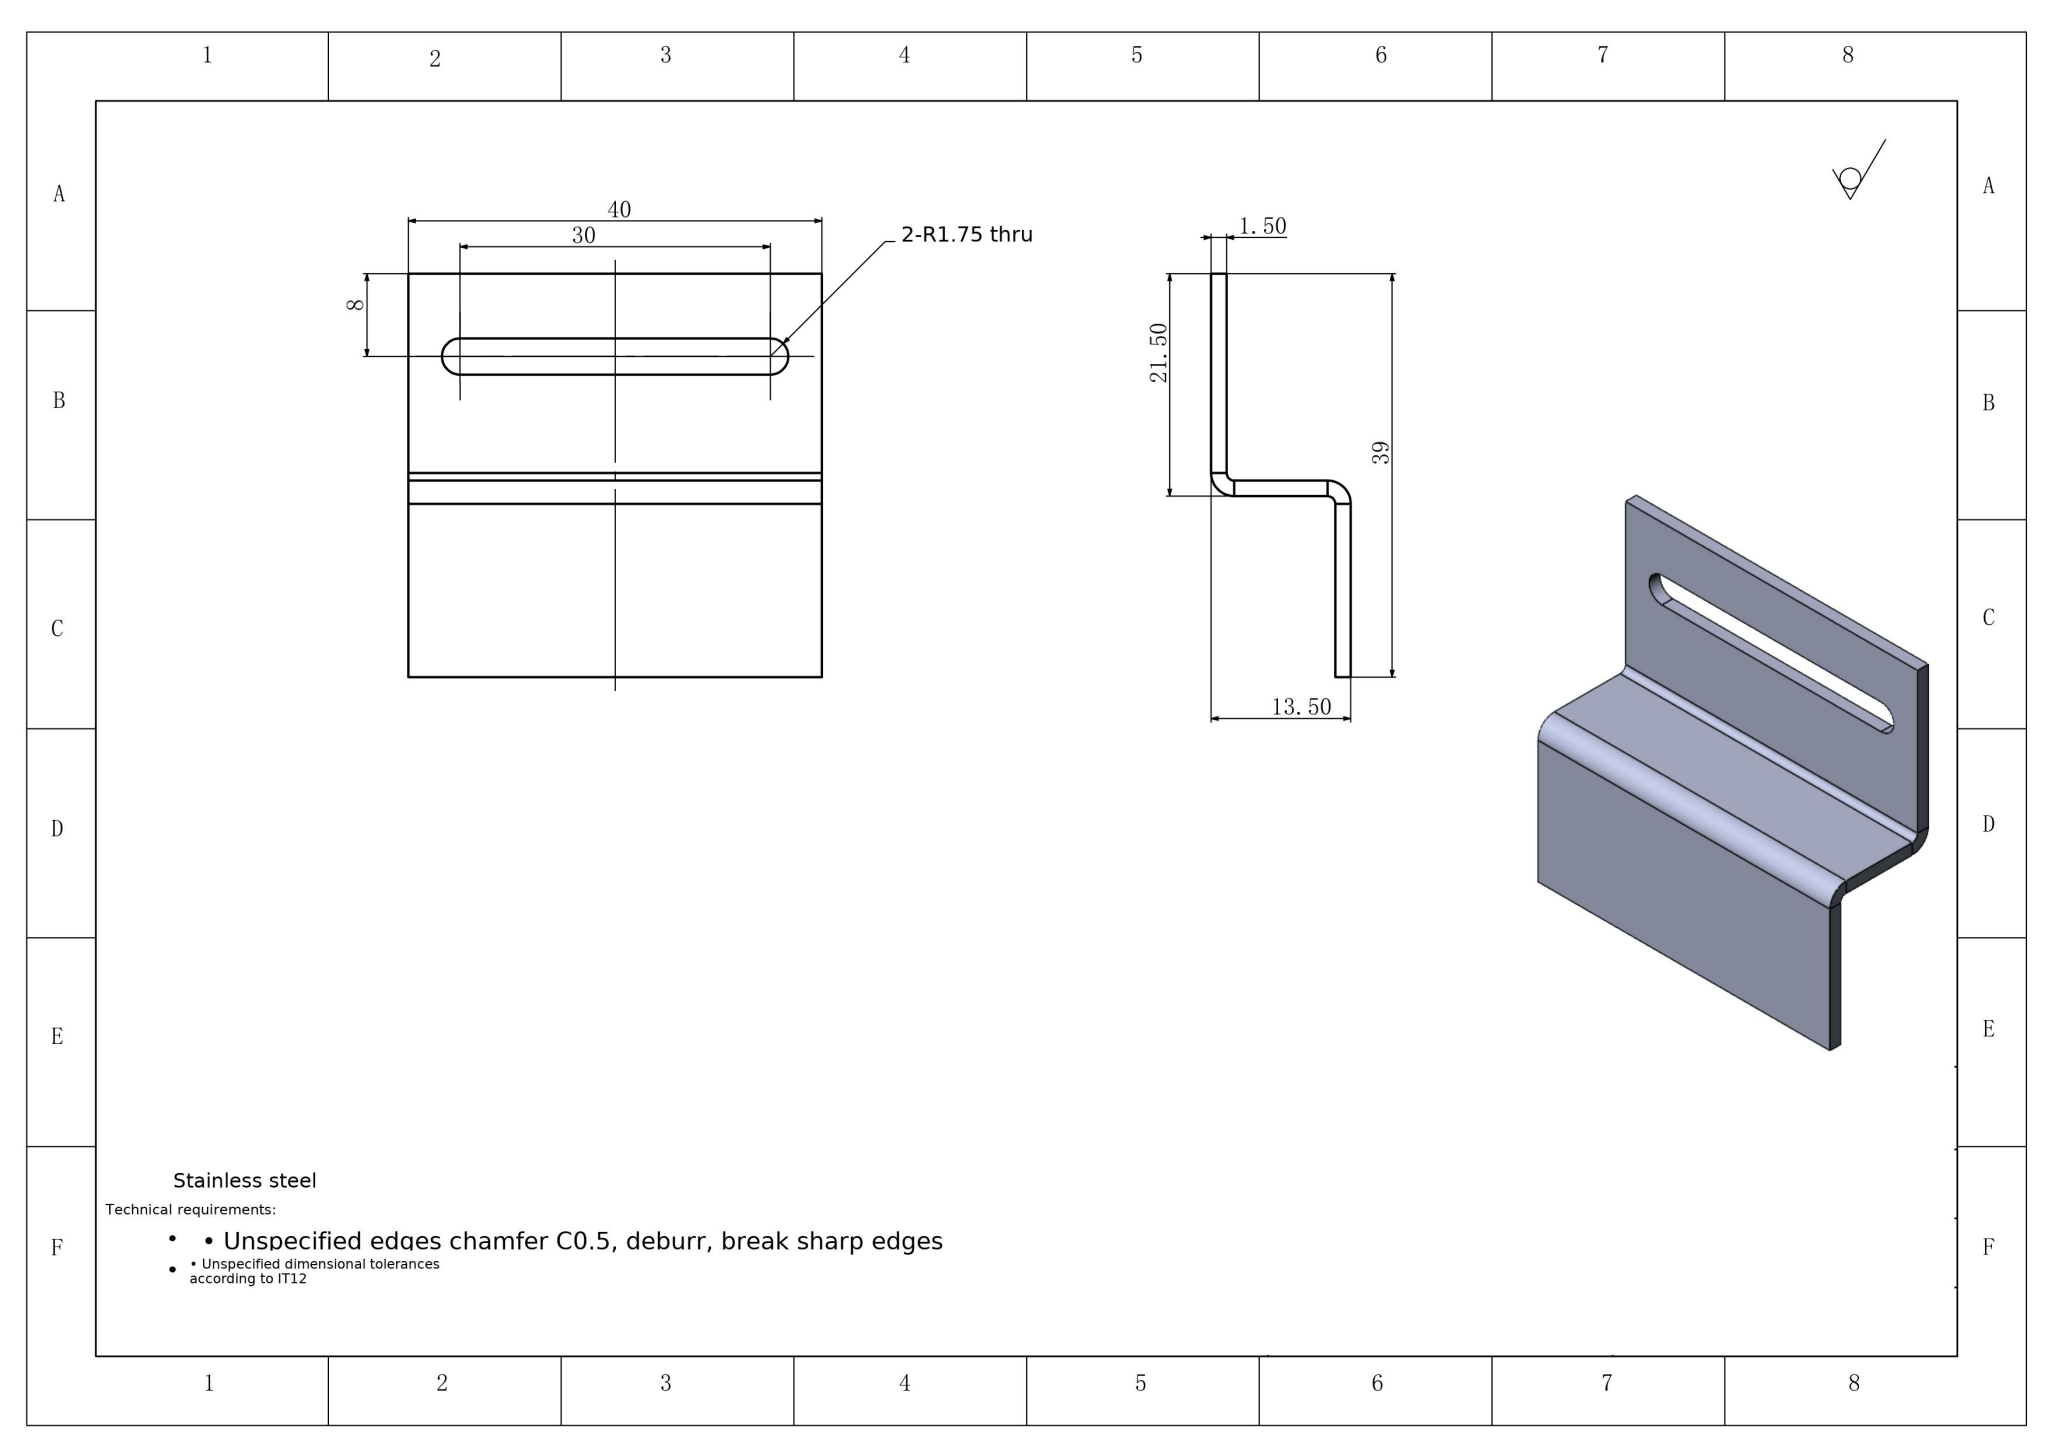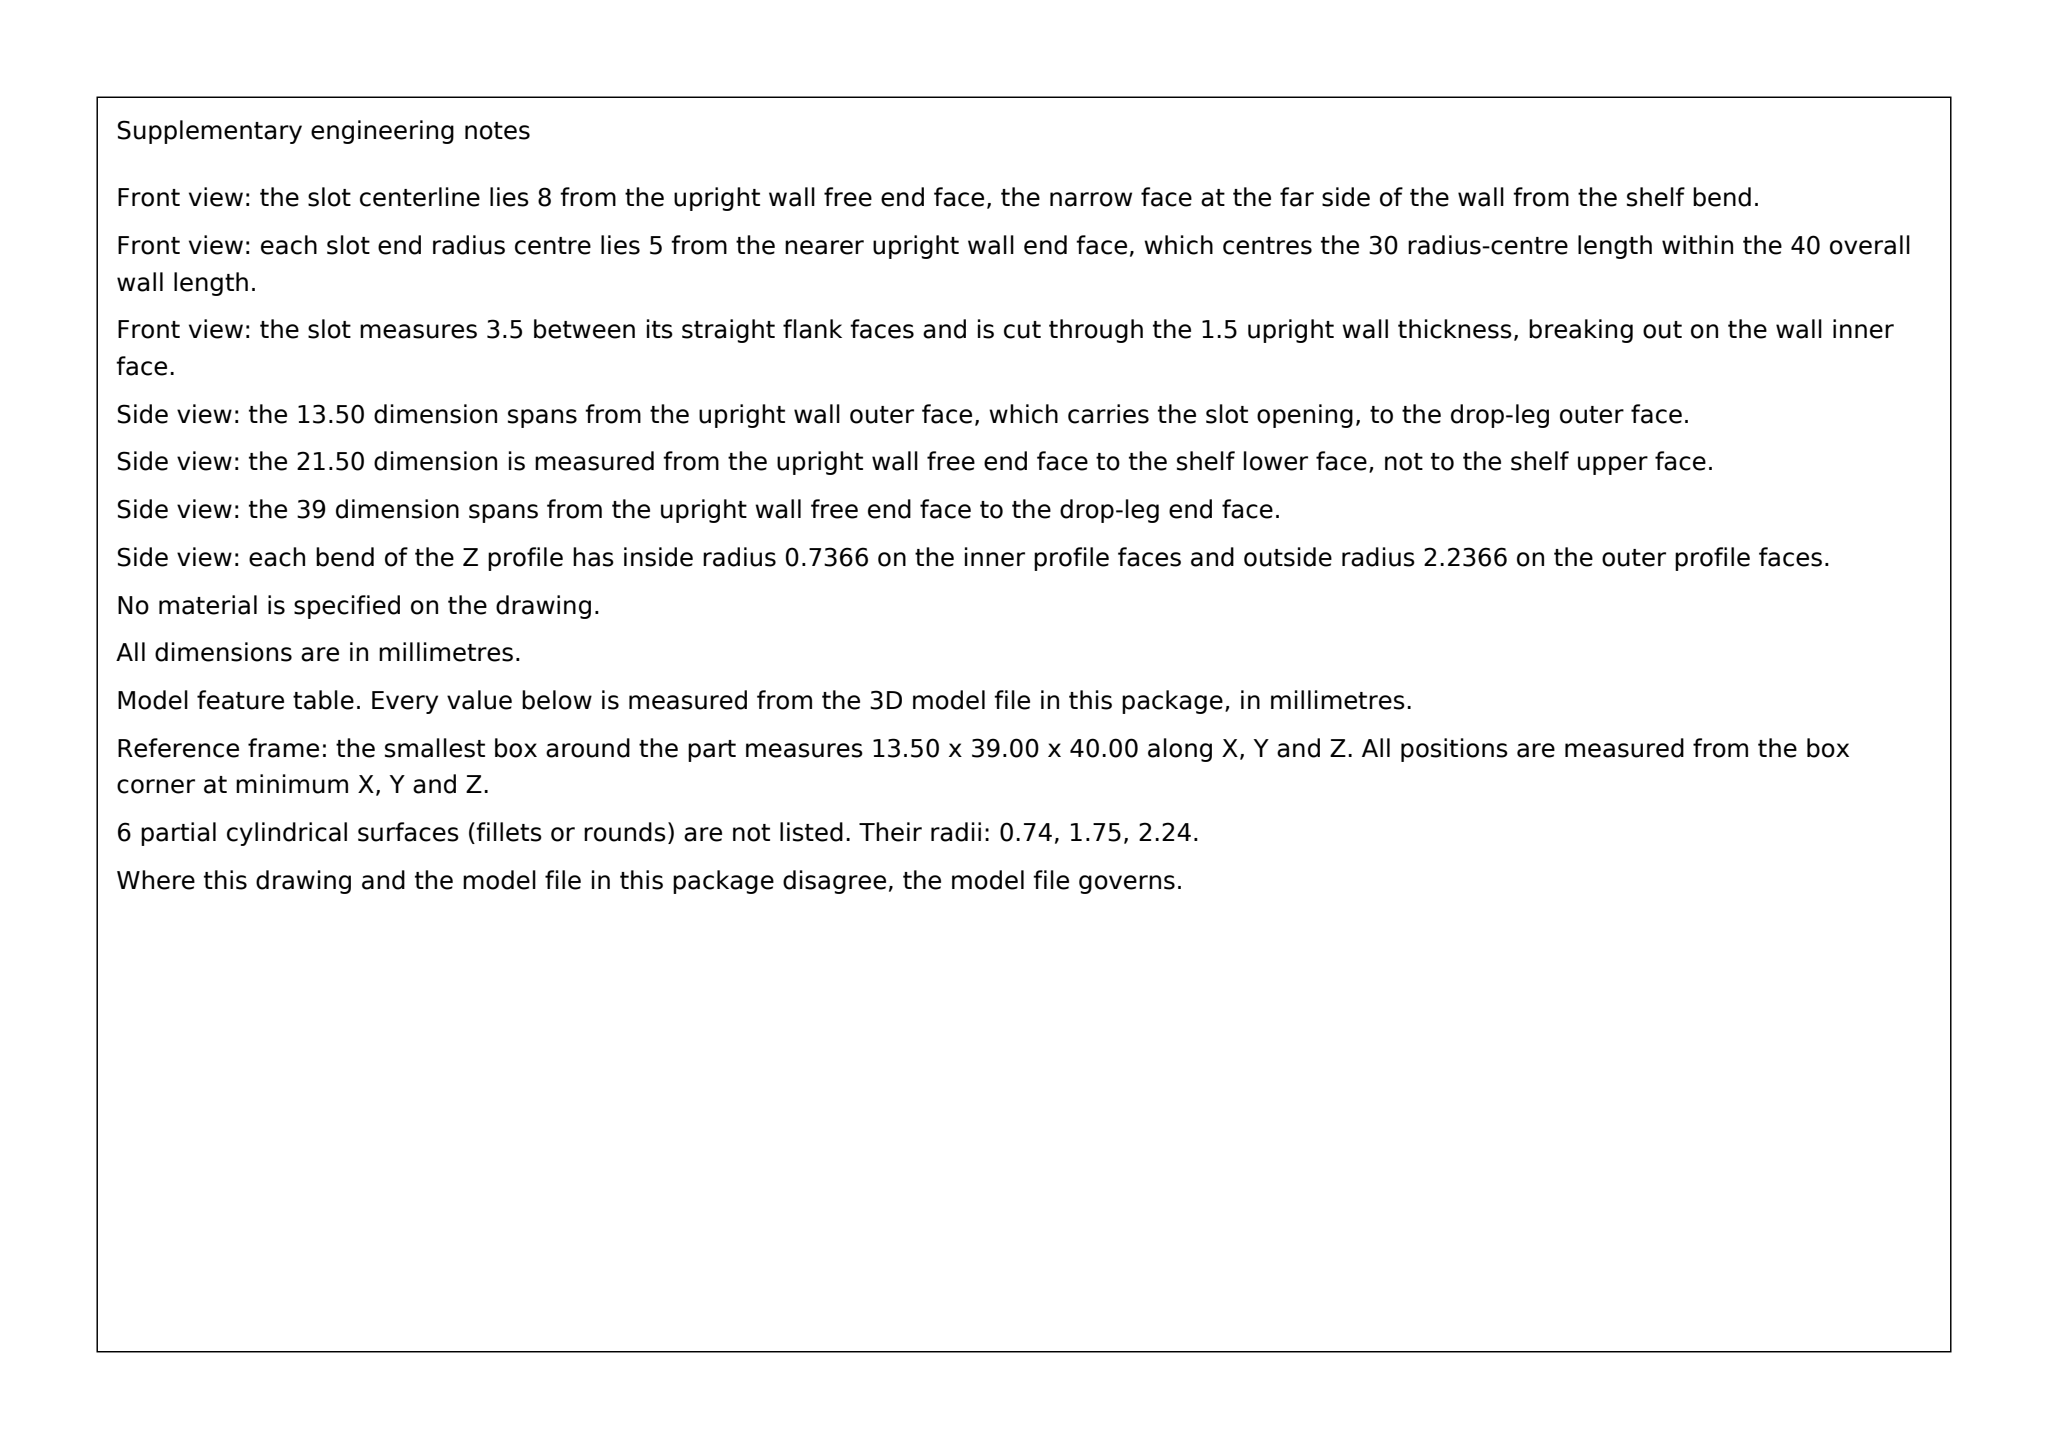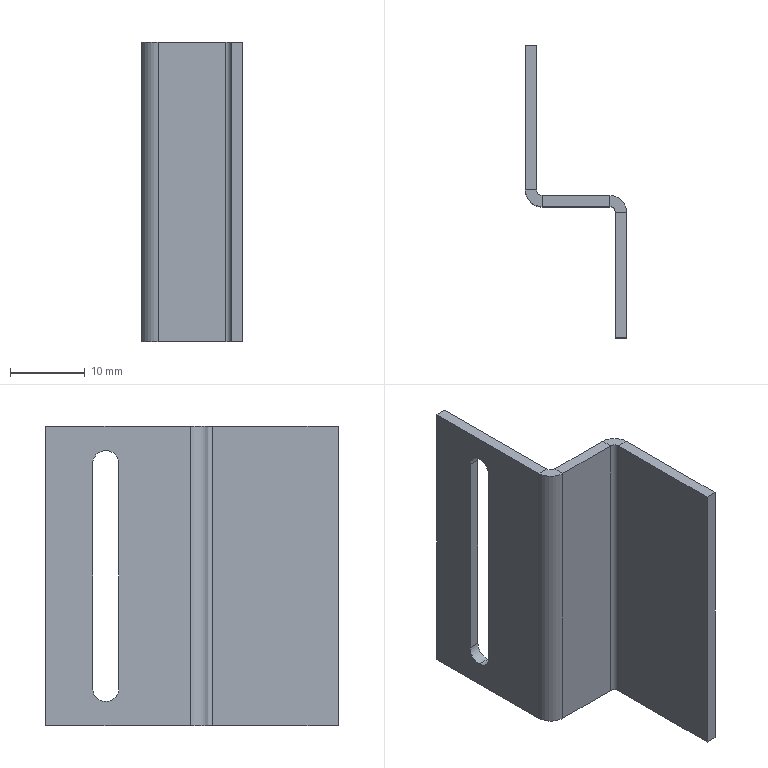Part | SolidWorks | mm | 1 solid | 27 faces | box 13.5 x 39 x 40 mm | volume 2812 mm3 | plane 20 | cylinder 7 | commonest cylinder face diameters 3.5 x3 4.473 x2 1.473 x2
Drawing notes:
ALL BENDS: INSIDE R0.74, OUTSIDE R2.24 (2 PLCS), T1.50 | from the solid: cylinders dia 1.473 (R0.737) & 4.473 (R2.237) about z at (2.24,19.74) and (11.26,16.76), L=40; wall planes x=0/1.5 give 1.5 thk
STEP:
#1=CARTESIAN_POINT('',(-1.5,12.,3.25));
#2=VERTEX_POINT('',#1);
#3=CARTESIAN_POINT('',(-1.5,13.75,5.));
#4=VERTEX_POINT('',#3);
#5=CARTESIAN_POINT('',(-1.5,12.,5.));
#6=DIRECTION('',(1.,0.,0.));
#7=DIRECTION('',(0.,0.,-1.));
#8=AXIS2_PLACEMENT_3D('',#5,#6,#7);
#9=CIRCLE('',#8,1.75);
#10=EDGE_CURVE('',#2,#4,#9,.T.);
#11=ORIENTED_EDGE('',*,*,#10,.F.);
#12=CARTESIAN_POINT('',(0.,12.,3.25));
#13=VERTEX_POINT('',#12);
#14=CARTESIAN_POINT('',(-1.5,12.,3.25));
#15=DIRECTION('',(1.,0.,0.));
#16=VECTOR('',#15,1000.);
#17=LINE('',#14,#16);
#18=EDGE_CURVE('',#2,#13,#17,.T.);
#19=ORIENTED_EDGE('',*,*,#18,.T.);
#20=CARTESIAN_POINT('',(0.,13.75,5.));
#21=VERTEX_POINT('',#20);
#22=CARTESIAN_POINT('',(0.,12.,5.));
#23=DIRECTION('',(1.,0.,0.));
#24=DIRECTION('',(0.,0.,-1.));
#25=AXIS2_PLACEMENT_3D('',#22,#23,#24);
#26=CIRCLE('',#25,1.75);
#27=EDGE_CURVE('',#13,#21,#26,.T.);
#28=ORIENTED_EDGE('',*,*,#27,.T.);
#29=CARTESIAN_POINT('',(-1.5,13.75,5.));
#30=DIRECTION('',(1.,0.,0.));
#31=VECTOR('',#30,1000.);
#32=LINE('',#29,#31);
#33=EDGE_CURVE('',#4,#21,#32,.T.);
#34=ORIENTED_EDGE('',*,*,#33,.F.);
#35=EDGE_LOOP('',(#11,#19,#28,#34));
#36=FACE_OUTER_BOUND('',#35,.T.);
#37=CARTESIAN_POINT('',(-1.5,12.,5.));
#38=DIRECTION('',(1.,0.,0.));
#39=DIRECTION('',(0.,0.,-1.));
#40=AXIS2_PLACEMENT_3D('',#37,#38,#39);
#41=CYLINDRICAL_SURFACE('',#40,1.75);
#42=ADVANCED_FACE('',(#36),#41,.F.);
#43=CARTESIAN_POINT('',(0.7366,0.,40.));
#44=VERTEX_POINT('',#43);
#45=CARTESIAN_POINT('',(0.7366,-1.5,40.));
#46=VERTEX_POINT('',#45);
#47=CARTESIAN_POINT('',(0.7366,0.,40.));
#48=DIRECTION('',(0.,-1.,0.));
#49=VECTOR('',#48,1000.);
#50=LINE('',#47,#49);
#51=EDGE_CURVE('',#44,#46,#50,.T.);
#52=ORIENTED_EDGE('',*,*,#51,.F.);
#53=CARTESIAN_POINT('',(0.,0.7366,40.));
#54=VERTEX_POINT('',#53);
#55=CARTESIAN_POINT('',(0.7366,0.7366,40.));
#56=DIRECTION('',(0.,0.,1.));
#57=DIRECTION('',(-1.,0.,0.));
#58=AXIS2_PLACEMENT_3D('',#55,#56,#57);
#59=CIRCLE('',#58,0.7366);
#60=EDGE_CURVE('',#54,#44,#59,.T.);
#61=ORIENTED_EDGE('',*,*,#60,.F.);
#62=CARTESIAN_POINT('',(-1.5,0.7366,40.));
#63=VERTEX_POINT('',#62);
#64=CARTESIAN_POINT('',(-1.5,0.7366,40.));
#65=DIRECTION('',(1.,-0.,0.));
#66=VECTOR('',#65,1000.);
#67=LINE('',#64,#66);
#68=EDGE_CURVE('',#63,#54,#67,.T.);
#69=ORIENTED_EDGE('',*,*,#68,.F.);
#70=CARTESIAN_POINT('',(0.7366,0.7366,40.));
#71=DIRECTION('',(0.,0.,1.));
#72=DIRECTION('',(1.,0.,0.));
#73=AXIS2_PLACEMENT_3D('',#70,#71,#72);
#74=CIRCLE('',#73,2.237);
#75=EDGE_CURVE('',#63,#46,#74,.T.);
#76=ORIENTED_EDGE('',*,*,#75,.T.);
#77=EDGE_LOOP('',(#52,#61,#69,#76));
#78=FACE_OUTER_BOUND('',#77,.T.);
#79=CARTESIAN_POINT('',(0.7366,0.,40.));
#80=DIRECTION('',(0.,0.,1.));
#81=DIRECTION('',(1.,0.,0.));
#82=AXIS2_PLACEMENT_3D('',#79,#80,#81);
#83=PLANE('',#82);
#84=ADVANCED_FACE('',(#78),#83,.T.);
#85=CARTESIAN_POINT('',(9.763,0.,40.));
#86=VERTEX_POINT('',#85);
#87=CARTESIAN_POINT('',(0.,0.,40.));
#88=DIRECTION('',(1.,0.,0.));
#89=VECTOR('',#88,1000.);
#90=LINE('',#87,#89);
#91=EDGE_CURVE('',#44,#86,#90,.T.);
#92=ORIENTED_EDGE('',*,*,#91,.F.);
#93=ORIENTED_EDGE('',*,*,#51,.T.);
#94=CARTESIAN_POINT('',(9.763,-1.5,40.));
#95=VERTEX_POINT('',#94);
#96=CARTESIAN_POINT('',(0.,-1.5,40.));
#97=DIRECTION('',(1.,0.,0.));
#98=VECTOR('',#97,1000.);
#99=LINE('',#96,#98);
#100=EDGE_CURVE('',#46,#95,#99,.T.);
#101=ORIENTED_EDGE('',*,*,#100,.T.);
#102=CARTESIAN_POINT('',(9.763,-1.5,40.));
#103=DIRECTION('',(0.,1.,0.));
#104=VECTOR('',#103,1000.);
#105=LINE('',#102,#104);
#106=EDGE_CURVE('',#95,#86,#105,.T.);
#107=ORIENTED_EDGE('',*,*,#106,.T.);
#108=EDGE_LOOP('',(#92,#93,#101,#107));
#109=FACE_OUTER_BOUND('',#108,.T.);
#110=CARTESIAN_POINT('',(-1.5,0.7366,40.));
#111=DIRECTION('',(0.,0.,1.));
#112=DIRECTION('',(1.,0.,0.));
#113=AXIS2_PLACEMENT_3D('',#110,#111,#112);
#114=PLANE('',#113);
#115=ADVANCED_FACE('',(#109),#114,.T.);
#116=CARTESIAN_POINT('',(0.,0.7366,0.));
#117=VERTEX_POINT('',#116);
#118=CARTESIAN_POINT('',(-1.5,0.7366,0.));
#119=VERTEX_POINT('',#118);
#120=CARTESIAN_POINT('',(0.,0.7366,0.));
#121=DIRECTION('',(-1.,0.,0.));
#122=VECTOR('',#121,1000.);
#123=LINE('',#120,#122);
#124=EDGE_CURVE('',#117,#119,#123,.T.);
#125=ORIENTED_EDGE('',*,*,#124,.F.);
#126=CARTESIAN_POINT('',(0.7366,0.,0.));
#127=VERTEX_POINT('',#126);
#128=CARTESIAN_POINT('',(0.7366,0.7366,0.));
#129=DIRECTION('',(0.,0.,1.));
#130=DIRECTION('',(-1.,0.,0.));
#131=AXIS2_PLACEMENT_3D('',#128,#129,#130);
#132=CIRCLE('',#131,0.7366);
#133=EDGE_CURVE('',#117,#127,#132,.T.);
#134=ORIENTED_EDGE('',*,*,#133,.T.);
#135=CARTESIAN_POINT('',(0.7366,-1.5,0.));
#136=VERTEX_POINT('',#135);
#137=CARTESIAN_POINT('',(0.7366,-1.5,0.));
#138=DIRECTION('',(0.,1.,0.));
#139=VECTOR('',#138,1000.);
#140=LINE('',#137,#139);
#141=EDGE_CURVE('',#136,#127,#140,.T.);
#142=ORIENTED_EDGE('',*,*,#141,.F.);
#143=CARTESIAN_POINT('',(0.7366,0.7366,0.));
#144=DIRECTION('',(0.,0.,1.));
#145=DIRECTION('',(1.,0.,0.));
#146=AXIS2_PLACEMENT_3D('',#143,#144,#145);
#147=CIRCLE('',#146,2.237);
#148=EDGE_CURVE('',#119,#136,#147,.T.);
#149=ORIENTED_EDGE('',*,*,#148,.F.);
#150=EDGE_LOOP('',(#125,#134,#142,#149));
#151=FACE_OUTER_BOUND('',#150,.T.);
#152=CARTESIAN_POINT('',(0.,0.7366,0.));
#153=DIRECTION('',(0.,0.,-1.));
#154=DIRECTION('',(-1.,0.,0.));
#155=AXIS2_PLACEMENT_3D('',#152,#153,#154);
#156=PLANE('',#155);
#157=ADVANCED_FACE('',(#151),#156,.T.);
#158=CARTESIAN_POINT('',(0.,20.,0.));
#159=VERTEX_POINT('',#158);
#160=CARTESIAN_POINT('',(0.,0.,0.));
#161=DIRECTION('',(0.,-1.,0.));
#162=VECTOR('',#161,1000.);
#163=LINE('',#160,#162);
#164=EDGE_CURVE('',#159,#117,#163,.T.);
#165=ORIENTED_EDGE('',*,*,#164,.T.);
#166=ORIENTED_EDGE('',*,*,#124,.T.);
#167=CARTESIAN_POINT('',(-1.5,20.,0.));
#168=VERTEX_POINT('',#167);
#169=CARTESIAN_POINT('',(-1.5,0.,0.));
#170=DIRECTION('',(0.,-1.,0.));
#171=VECTOR('',#170,1000.);
#172=LINE('',#169,#171);
#173=EDGE_CURVE('',#168,#119,#172,.T.);
#174=ORIENTED_EDGE('',*,*,#173,.F.);
#175=CARTESIAN_POINT('',(-1.5,20.,0.));
#176=DIRECTION('',(1.,0.,0.));
#177=VECTOR('',#176,1000.);
#178=LINE('',#175,#177);
#179=EDGE_CURVE('',#168,#159,#178,.T.);
#180=ORIENTED_EDGE('',*,*,#179,.T.);
#181=EDGE_LOOP('',(#165,#166,#174,#180));
#182=FACE_OUTER_BOUND('',#181,.T.);
#183=CARTESIAN_POINT('',(0.7366,-1.5,0.));
#184=DIRECTION('',(0.,0.,-1.));
#185=DIRECTION('',(-1.,0.,0.));
#186=AXIS2_PLACEMENT_3D('',#183,#184,#185);
#187=PLANE('',#186);
#188=ADVANCED_FACE('',(#182),#187,.T.);
#189=CARTESIAN_POINT('',(12.,-2.237,40.));
#190=VERTEX_POINT('',#189);
#191=CARTESIAN_POINT('',(10.5,-2.237,40.));
#192=VERTEX_POINT('',#191);
#193=CARTESIAN_POINT('',(12.,-2.237,40.));
#194=DIRECTION('',(-1.,0.,0.));
#195=VECTOR('',#194,1000.);
#196=LINE('',#193,#195);
#197=EDGE_CURVE('',#190,#192,#196,.T.);
#198=ORIENTED_EDGE('',*,*,#197,.F.);
#199=CARTESIAN_POINT('',(9.763,-2.237,40.));
#200=DIRECTION('',(0.,0.,-1.));
#201=DIRECTION('',(1.,0.,0.));
#202=AXIS2_PLACEMENT_3D('',#199,#200,#201);
#203=CIRCLE('',#202,2.237);
#204=EDGE_CURVE('',#86,#190,#203,.T.);
#205=ORIENTED_EDGE('',*,*,#204,.F.);
#206=ORIENTED_EDGE('',*,*,#106,.F.);
#207=CARTESIAN_POINT('',(9.763,-2.237,40.));
#208=DIRECTION('',(0.,0.,-1.));
#209=DIRECTION('',(1.,0.,0.));
#210=AXIS2_PLACEMENT_3D('',#207,#208,#209);
#211=CIRCLE('',#210,0.7366);
#212=EDGE_CURVE('',#95,#192,#211,.T.);
#213=ORIENTED_EDGE('',*,*,#212,.T.);
#214=EDGE_LOOP('',(#198,#205,#206,#213));
#215=FACE_OUTER_BOUND('',#214,.T.);
#216=CARTESIAN_POINT('',(12.,-2.237,40.));
#217=DIRECTION('',(0.,0.,1.));
#218=DIRECTION('',(1.,0.,0.));
#219=AXIS2_PLACEMENT_3D('',#216,#217,#218);
#220=PLANE('',#219);
#221=ADVANCED_FACE('',(#215),#220,.T.);
#222=CARTESIAN_POINT('',(12.,-19.,40.));
#223=VERTEX_POINT('',#222);
#224=CARTESIAN_POINT('',(12.,0.,40.));
#225=DIRECTION('',(0.,-1.,0.));
#226=VECTOR('',#225,1000.);
#227=LINE('',#224,#226);
#228=EDGE_CURVE('',#190,#223,#227,.T.);
#229=ORIENTED_EDGE('',*,*,#228,.F.);
#230=ORIENTED_EDGE('',*,*,#197,.T.);
#231=CARTESIAN_POINT('',(10.5,-19.,40.));
#232=VERTEX_POINT('',#231);
#233=CARTESIAN_POINT('',(10.5,-0.,40.));
#234=DIRECTION('',(0.,-1.,0.));
#235=VECTOR('',#234,1000.);
#236=LINE('',#233,#235);
#237=EDGE_CURVE('',#192,#232,#236,.T.);
#238=ORIENTED_EDGE('',*,*,#237,.T.);
#239=CARTESIAN_POINT('',(12.,-19.,40.));
#240=DIRECTION('',(-1.,0.,0.));
#241=VECTOR('',#240,1000.);
#242=LINE('',#239,#241);
#243=EDGE_CURVE('',#223,#232,#242,.T.);
#244=ORIENTED_EDGE('',*,*,#243,.F.);
#245=EDGE_LOOP('',(#229,#230,#238,#244));
#246=FACE_OUTER_BOUND('',#245,.T.);
#247=CARTESIAN_POINT('',(9.763,-1.5,40.));
#248=DIRECTION('',(0.,0.,1.));
#249=DIRECTION('',(1.,0.,0.));
#250=AXIS2_PLACEMENT_3D('',#247,#248,#249);
#251=PLANE('',#250);
#252=ADVANCED_FACE('',(#246),#251,.T.);
#253=CARTESIAN_POINT('',(9.763,0.,0.));
#254=VERTEX_POINT('',#253);
#255=CARTESIAN_POINT('',(9.763,-1.5,0.));
#256=VERTEX_POINT('',#255);
#257=CARTESIAN_POINT('',(9.763,0.,0.));
#258=DIRECTION('',(0.,-1.,0.));
#259=VECTOR('',#258,1000.);
#260=LINE('',#257,#259);
#261=EDGE_CURVE('',#254,#256,#260,.T.);
#262=ORIENTED_EDGE('',*,*,#261,.F.);
#263=CARTESIAN_POINT('',(12.,-2.237,0.));
#264=VERTEX_POINT('',#263);
#265=CARTESIAN_POINT('',(9.763,-2.237,0.));
#266=DIRECTION('',(0.,0.,-1.));
#267=DIRECTION('',(1.,0.,0.));
#268=AXIS2_PLACEMENT_3D('',#265,#266,#267);
#269=CIRCLE('',#268,2.237);
#270=EDGE_CURVE('',#254,#264,#269,.T.);
#271=ORIENTED_EDGE('',*,*,#270,.T.);
#272=CARTESIAN_POINT('',(10.5,-2.237,0.));
#273=VERTEX_POINT('',#272);
#274=CARTESIAN_POINT('',(10.5,-2.237,0.));
#275=DIRECTION('',(1.,0.,0.));
#276=VECTOR('',#275,1000.);
#277=LINE('',#274,#276);
#278=EDGE_CURVE('',#273,#264,#277,.T.);
#279=ORIENTED_EDGE('',*,*,#278,.F.);
#280=CARTESIAN_POINT('',(9.763,-2.237,0.));
#281=DIRECTION('',(0.,0.,-1.));
#282=DIRECTION('',(1.,0.,0.));
#283=AXIS2_PLACEMENT_3D('',#280,#281,#282);
#284=CIRCLE('',#283,0.7366);
#285=EDGE_CURVE('',#256,#273,#284,.T.);
#286=ORIENTED_EDGE('',*,*,#285,.F.);
#287=EDGE_LOOP('',(#262,#271,#279,#286));
#288=FACE_OUTER_BOUND('',#287,.T.);
#289=CARTESIAN_POINT('',(9.763,0.,0.));
#290=DIRECTION('',(0.,0.,-1.));
#291=DIRECTION('',(-1.,0.,0.));
#292=AXIS2_PLACEMENT_3D('',#289,#290,#291);
#293=PLANE('',#292);
#294=ADVANCED_FACE('',(#288),#293,.T.);
#295=CARTESIAN_POINT('',(0.,0.,0.));
#296=DIRECTION('',(1.,0.,0.));
#297=VECTOR('',#296,1000.);
#298=LINE('',#295,#297);
#299=EDGE_CURVE('',#127,#254,#298,.T.);
#300=ORIENTED_EDGE('',*,*,#299,.T.);
#301=ORIENTED_EDGE('',*,*,#261,.T.);
#302=CARTESIAN_POINT('',(0.,-1.5,0.));
#303=DIRECTION('',(1.,0.,0.));
#304=VECTOR('',#303,1000.);
#305=LINE('',#302,#304);
#306=EDGE_CURVE('',#136,#256,#305,.T.);
#307=ORIENTED_EDGE('',*,*,#306,.F.);
#308=ORIENTED_EDGE('',*,*,#141,.T.);
#309=EDGE_LOOP('',(#300,#301,#307,#308));
#310=FACE_OUTER_BOUND('',#309,.T.);
#311=CARTESIAN_POINT('',(10.5,-2.237,0.));
#312=DIRECTION('',(0.,0.,-1.));
#313=DIRECTION('',(-1.,0.,0.));
#314=AXIS2_PLACEMENT_3D('',#311,#312,#313);
#315=PLANE('',#314);
#316=ADVANCED_FACE('',(#310),#315,.T.);
#317=CARTESIAN_POINT('',(10.5,-19.,0.));
#318=VERTEX_POINT('',#317);
#319=CARTESIAN_POINT('',(10.5,-0.,0.));
#320=DIRECTION('',(0.,-1.,0.));
#321=VECTOR('',#320,1000.);
#322=LINE('',#319,#321);
#323=EDGE_CURVE('',#273,#318,#322,.T.);
#324=ORIENTED_EDGE('',*,*,#323,.T.);
#325=CARTESIAN_POINT('',(10.5,-19.,40.));
#326=DIRECTION('',(0.,0.,-1.));
#327=VECTOR('',#326,1000.);
#328=LINE('',#325,#327);
#329=EDGE_CURVE('',#232,#318,#328,.T.);
#330=ORIENTED_EDGE('',*,*,#329,.F.);
#331=ORIENTED_EDGE('',*,*,#237,.F.);
#332=CARTESIAN_POINT('',(10.5,-2.237,40.));
#333=DIRECTION('',(0.,0.,-1.));
#334=VECTOR('',#333,1000.);
#335=LINE('',#332,#334);
#336=EDGE_CURVE('',#192,#273,#335,.T.);
#337=ORIENTED_EDGE('',*,*,#336,.T.);
#338=EDGE_LOOP('',(#324,#330,#331,#337));
#339=FACE_OUTER_BOUND('',#338,.T.);
#340=CARTESIAN_POINT('',(10.5,-0.,40.));
#341=DIRECTION('',(1.,0.,0.));
#342=DIRECTION('',(-0.,1.,0.));
#343=AXIS2_PLACEMENT_3D('',#340,#341,#342);
#344=PLANE('',#343);
#345=ADVANCED_FACE('',(#339),#344,.F.);
#346=CARTESIAN_POINT('',(12.,-19.,0.));
#347=VERTEX_POINT('',#346);
#348=CARTESIAN_POINT('',(12.,-19.,0.));
#349=DIRECTION('',(-1.,0.,0.));
#350=VECTOR('',#349,1000.);
#351=LINE('',#348,#350);
#352=EDGE_CURVE('',#347,#318,#351,.T.);
#353=ORIENTED_EDGE('',*,*,#352,.F.);
#354=CARTESIAN_POINT('',(12.,-19.,40.));
#355=DIRECTION('',(0.,0.,-1.));
#356=VECTOR('',#355,1000.);
#357=LINE('',#354,#356);
#358=EDGE_CURVE('',#223,#347,#357,.T.);
#359=ORIENTED_EDGE('',*,*,#358,.F.);
#360=ORIENTED_EDGE('',*,*,#243,.T.);
#361=ORIENTED_EDGE('',*,*,#329,.T.);
#362=EDGE_LOOP('',(#353,#359,#360,#361));
#363=FACE_OUTER_BOUND('',#362,.T.);
#364=CARTESIAN_POINT('',(12.,-19.,40.));
#365=DIRECTION('',(0.,-1.,0.));
#366=DIRECTION('',(0.,0.,-1.));
#367=AXIS2_PLACEMENT_3D('',#364,#365,#366);
#368=PLANE('',#367);
#369=ADVANCED_FACE('',(#363),#368,.T.);
#370=CARTESIAN_POINT('',(12.,0.,0.));
#371=DIRECTION('',(0.,-1.,0.));
#372=VECTOR('',#371,1000.);
#373=LINE('',#370,#372);
#374=EDGE_CURVE('',#264,#347,#373,.T.);
#375=ORIENTED_EDGE('',*,*,#374,.F.);
#376=CARTESIAN_POINT('',(12.,-2.237,40.));
#377=DIRECTION('',(0.,0.,-1.));
#378=VECTOR('',#377,1000.);
#379=LINE('',#376,#378);
#380=EDGE_CURVE('',#190,#264,#379,.T.);
#381=ORIENTED_EDGE('',*,*,#380,.F.);
#382=ORIENTED_EDGE('',*,*,#228,.T.);
#383=ORIENTED_EDGE('',*,*,#358,.T.);
#384=EDGE_LOOP('',(#375,#381,#382,#383));
#385=FACE_OUTER_BOUND('',#384,.T.);
#386=CARTESIAN_POINT('',(12.,0.,40.));
#387=DIRECTION('',(1.,0.,0.));
#388=DIRECTION('',(-0.,1.,0.));
#389=AXIS2_PLACEMENT_3D('',#386,#387,#388);
#390=PLANE('',#389);
#391=ADVANCED_FACE('',(#385),#390,.T.);
#392=ORIENTED_EDGE('',*,*,#270,.F.);
#393=CARTESIAN_POINT('',(9.763,0.,40.));
#394=DIRECTION('',(0.,0.,-1.));
#395=VECTOR('',#394,1000.);
#396=LINE('',#393,#395);
#397=EDGE_CURVE('',#86,#254,#396,.T.);
#398=ORIENTED_EDGE('',*,*,#397,.F.);
#399=ORIENTED_EDGE('',*,*,#204,.T.);
#400=ORIENTED_EDGE('',*,*,#380,.T.);
#401=EDGE_LOOP('',(#392,#398,#399,#400));
#402=FACE_OUTER_BOUND('',#401,.T.);
#403=CARTESIAN_POINT('',(9.763,-2.237,40.));
#404=DIRECTION('',(0.,0.,-1.));
#405=DIRECTION('',(-1.,0.,0.));
#406=AXIS2_PLACEMENT_3D('',#403,#404,#405);
#407=CYLINDRICAL_SURFACE('',#406,2.237);
#408=ADVANCED_FACE('',(#402),#407,.T.);
#409=ORIENTED_EDGE('',*,*,#299,.F.);
#410=CARTESIAN_POINT('',(0.7366,0.,40.));
#411=DIRECTION('',(0.,0.,-1.));
#412=VECTOR('',#411,1000.);
#413=LINE('',#410,#412);
#414=EDGE_CURVE('',#44,#127,#413,.T.);
#415=ORIENTED_EDGE('',*,*,#414,.F.);
#416=ORIENTED_EDGE('',*,*,#91,.T.);
#417=ORIENTED_EDGE('',*,*,#397,.T.);
#418=EDGE_LOOP('',(#409,#415,#416,#417));
#419=FACE_OUTER_BOUND('',#418,.T.);
#420=CARTESIAN_POINT('',(0.,0.,40.));
#421=DIRECTION('',(0.,1.,0.));
#422=DIRECTION('',(0.,0.,1.));
#423=AXIS2_PLACEMENT_3D('',#420,#421,#422);
#424=PLANE('',#423);
#425=ADVANCED_FACE('',(#419),#424,.T.);
#426=ORIENTED_EDGE('',*,*,#133,.F.);
#427=CARTESIAN_POINT('',(0.,0.7366,40.));
#428=DIRECTION('',(0.,0.,-1.));
#429=VECTOR('',#428,1000.);
#430=LINE('',#427,#429);
#431=EDGE_CURVE('',#54,#117,#430,.T.);
#432=ORIENTED_EDGE('',*,*,#431,.F.);
#433=ORIENTED_EDGE('',*,*,#60,.T.);
#434=ORIENTED_EDGE('',*,*,#414,.T.);
#435=EDGE_LOOP('',(#426,#432,#433,#434));
#436=FACE_OUTER_BOUND('',#435,.T.);
#437=CARTESIAN_POINT('',(0.7366,0.7366,40.));
#438=DIRECTION('',(0.,0.,-1.));
#439=DIRECTION('',(-1.,0.,0.));
#440=AXIS2_PLACEMENT_3D('',#437,#438,#439);
#441=CYLINDRICAL_SURFACE('',#440,0.7366);
#442=ADVANCED_FACE('',(#436),#441,.F.);
#443=CARTESIAN_POINT('',(0.,13.75,35.));
#444=VERTEX_POINT('',#443);
#445=CARTESIAN_POINT('',(0.,10.25,35.));
#446=VERTEX_POINT('',#445);
#447=CARTESIAN_POINT('',(0.,12.,35.));
#448=DIRECTION('',(1.,0.,0.));
#449=DIRECTION('',(0.,0.,-1.));
#450=AXIS2_PLACEMENT_3D('',#447,#448,#449);
#451=CIRCLE('',#450,1.75);
#452=EDGE_CURVE('',#444,#446,#451,.T.);
#453=ORIENTED_EDGE('',*,*,#452,.F.);
#454=CARTESIAN_POINT('',(0.,13.75,35.));
#455=DIRECTION('',(0.,-0.,1.));
#456=VECTOR('',#455,1000.);
#457=LINE('',#454,#456);
#458=EDGE_CURVE('',#21,#444,#457,.T.);
#459=ORIENTED_EDGE('',*,*,#458,.F.);
#460=ORIENTED_EDGE('',*,*,#27,.F.);
#461=CARTESIAN_POINT('',(0.,10.25,5.));
#462=VERTEX_POINT('',#461);
#463=CARTESIAN_POINT('',(0.,12.,5.));
#464=DIRECTION('',(1.,0.,0.));
#465=DIRECTION('',(0.,0.,-1.));
#466=AXIS2_PLACEMENT_3D('',#463,#464,#465);
#467=CIRCLE('',#466,1.75);
#468=EDGE_CURVE('',#462,#13,#467,.T.);
#469=ORIENTED_EDGE('',*,*,#468,.F.);
#470=CARTESIAN_POINT('',(0.,10.25,35.));
#471=DIRECTION('',(0.,0.,-1.));
#472=VECTOR('',#471,1000.);
#473=LINE('',#470,#472);
#474=EDGE_CURVE('',#446,#462,#473,.T.);
#475=ORIENTED_EDGE('',*,*,#474,.F.);
#476=EDGE_LOOP('',(#453,#459,#460,#469,#475));
#477=FACE_BOUND('',#476,.T.);
#478=ORIENTED_EDGE('',*,*,#164,.F.);
#479=CARTESIAN_POINT('',(0.,20.,40.));
#480=VERTEX_POINT('',#479);
#481=CARTESIAN_POINT('',(0.,20.,40.));
#482=DIRECTION('',(0.,0.,-1.));
#483=VECTOR('',#482,1000.);
#484=LINE('',#481,#483);
#485=EDGE_CURVE('',#480,#159,#484,.T.);
#486=ORIENTED_EDGE('',*,*,#485,.F.);
#487=CARTESIAN_POINT('',(0.,0.,40.));
#488=DIRECTION('',(0.,-1.,0.));
#489=VECTOR('',#488,1000.);
#490=LINE('',#487,#489);
#491=EDGE_CURVE('',#480,#54,#490,.T.);
#492=ORIENTED_EDGE('',*,*,#491,.T.);
#493=ORIENTED_EDGE('',*,*,#431,.T.);
#494=EDGE_LOOP('',(#478,#486,#492,#493));
#495=FACE_OUTER_BOUND('',#494,.T.);
#496=CARTESIAN_POINT('',(0.,0.,40.));
#497=DIRECTION('',(1.,0.,0.));
#498=DIRECTION('',(0.,0.,-1.));
#499=AXIS2_PLACEMENT_3D('',#496,#497,#498);
#500=PLANE('',#499);
#501=ADVANCED_FACE('',(#477,#495),#500,.T.);
#502=ORIENTED_EDGE('',*,*,#179,.F.);
#503=CARTESIAN_POINT('',(-1.5,20.,40.));
#504=VERTEX_POINT('',#503);
#505=CARTESIAN_POINT('',(-1.5,20.,40.));
#506=DIRECTION('',(0.,0.,-1.));
#507=VECTOR('',#506,1000.);
#508=LINE('',#505,#507);
#509=EDGE_CURVE('',#504,#168,#508,.T.);
#510=ORIENTED_EDGE('',*,*,#509,.F.);
#511=CARTESIAN_POINT('',(-1.5,20.,40.));
#512=DIRECTION('',(1.,0.,0.));
#513=VECTOR('',#512,1000.);
#514=LINE('',#511,#513);
#515=EDGE_CURVE('',#504,#480,#514,.T.);
#516=ORIENTED_EDGE('',*,*,#515,.T.);
#517=ORIENTED_EDGE('',*,*,#485,.T.);
#518=EDGE_LOOP('',(#502,#510,#516,#517));
#519=FACE_OUTER_BOUND('',#518,.T.);
#520=CARTESIAN_POINT('',(-1.5,20.,40.));
#521=DIRECTION('',(0.,1.,0.));
#522=DIRECTION('',(0.,0.,1.));
#523=AXIS2_PLACEMENT_3D('',#520,#521,#522);
#524=PLANE('',#523);
#525=ADVANCED_FACE('',(#519),#524,.T.);
#526=CARTESIAN_POINT('',(-1.5,13.75,35.));
#527=VERTEX_POINT('',#526);
#528=CARTESIAN_POINT('',(-1.5,13.75,35.));
#529=DIRECTION('',(0.,-0.,1.));
#530=VECTOR('',#529,1000.);
#531=LINE('',#528,#530);
#532=EDGE_CURVE('',#4,#527,#531,.T.);
#533=ORIENTED_EDGE('',*,*,#532,.T.);
#534=CARTESIAN_POINT('',(-1.5,10.25,35.));
#535=VERTEX_POINT('',#534);
#536=CARTESIAN_POINT('',(-1.5,12.,35.));
#537=DIRECTION('',(1.,0.,0.));
#538=DIRECTION('',(0.,0.,-1.));
#539=AXIS2_PLACEMENT_3D('',#536,#537,#538);
#540=CIRCLE('',#539,1.75);
#541=EDGE_CURVE('',#527,#535,#540,.T.);
#542=ORIENTED_EDGE('',*,*,#541,.T.);
#543=CARTESIAN_POINT('',(-1.5,10.25,5.));
#544=VERTEX_POINT('',#543);
#545=CARTESIAN_POINT('',(-1.5,10.25,35.));
#546=DIRECTION('',(0.,0.,-1.));
#547=VECTOR('',#546,1000.);
#548=LINE('',#545,#547);
#549=EDGE_CURVE('',#535,#544,#548,.T.);
#550=ORIENTED_EDGE('',*,*,#549,.T.);
#551=CARTESIAN_POINT('',(-1.5,12.,5.));
#552=DIRECTION('',(1.,0.,0.));
#553=DIRECTION('',(0.,0.,-1.));
#554=AXIS2_PLACEMENT_3D('',#551,#552,#553);
#555=CIRCLE('',#554,1.75);
#556=EDGE_CURVE('',#544,#2,#555,.T.);
#557=ORIENTED_EDGE('',*,*,#556,.T.);
#558=ORIENTED_EDGE('',*,*,#10,.T.);
#559=EDGE_LOOP('',(#533,#542,#550,#557,#558));
#560=FACE_BOUND('',#559,.T.);
#561=ORIENTED_EDGE('',*,*,#173,.T.);
#562=CARTESIAN_POINT('',(-1.5,0.7366,40.));
#563=DIRECTION('',(0.,0.,-1.));
#564=VECTOR('',#563,1000.);
#565=LINE('',#562,#564);
#566=EDGE_CURVE('',#63,#119,#565,.T.);
#567=ORIENTED_EDGE('',*,*,#566,.F.);
#568=CARTESIAN_POINT('',(-1.5,0.,40.));
#569=DIRECTION('',(0.,-1.,0.));
#570=VECTOR('',#569,1000.);
#571=LINE('',#568,#570);
#572=EDGE_CURVE('',#504,#63,#571,.T.);
#573=ORIENTED_EDGE('',*,*,#572,.F.);
#574=ORIENTED_EDGE('',*,*,#509,.T.);
#575=EDGE_LOOP('',(#561,#567,#573,#574));
#576=FACE_OUTER_BOUND('',#575,.T.);
#577=CARTESIAN_POINT('',(-1.5,0.,40.));
#578=DIRECTION('',(1.,0.,0.));
#579=DIRECTION('',(0.,0.,-1.));
#580=AXIS2_PLACEMENT_3D('',#577,#578,#579);
#581=PLANE('',#580);
#582=ADVANCED_FACE('',(#560,#576),#581,.F.);
#583=ORIENTED_EDGE('',*,*,#148,.T.);
#584=CARTESIAN_POINT('',(0.7366,-1.5,40.));
#585=DIRECTION('',(0.,0.,-1.));
#586=VECTOR('',#585,1000.);
#587=LINE('',#584,#586);
#588=EDGE_CURVE('',#46,#136,#587,.T.);
#589=ORIENTED_EDGE('',*,*,#588,.F.);
#590=ORIENTED_EDGE('',*,*,#75,.F.);
#591=ORIENTED_EDGE('',*,*,#566,.T.);
#592=EDGE_LOOP('',(#583,#589,#590,#591));
#593=FACE_OUTER_BOUND('',#592,.T.);
#594=CARTESIAN_POINT('',(0.7366,0.7366,40.));
#595=DIRECTION('',(0.,0.,-1.));
#596=DIRECTION('',(-1.,0.,0.));
#597=AXIS2_PLACEMENT_3D('',#594,#595,#596);
#598=CYLINDRICAL_SURFACE('',#597,2.237);
#599=ADVANCED_FACE('',(#593),#598,.T.);
#600=ORIENTED_EDGE('',*,*,#306,.T.);
#601=CARTESIAN_POINT('',(9.763,-1.5,40.));
#602=DIRECTION('',(0.,0.,-1.));
#603=VECTOR('',#602,1000.);
#604=LINE('',#601,#603);
#605=EDGE_CURVE('',#95,#256,#604,.T.);
#606=ORIENTED_EDGE('',*,*,#605,.F.);
#607=ORIENTED_EDGE('',*,*,#100,.F.);
#608=ORIENTED_EDGE('',*,*,#588,.T.);
#609=EDGE_LOOP('',(#600,#606,#607,#608));
#610=FACE_OUTER_BOUND('',#609,.T.);
#611=CARTESIAN_POINT('',(0.,-1.5,40.));
#612=DIRECTION('',(0.,1.,0.));
#613=DIRECTION('',(0.,0.,1.));
#614=AXIS2_PLACEMENT_3D('',#611,#612,#613);
#615=PLANE('',#614);
#616=ADVANCED_FACE('',(#610),#615,.F.);
#617=ORIENTED_EDGE('',*,*,#285,.T.);
#618=ORIENTED_EDGE('',*,*,#336,.F.);
#619=ORIENTED_EDGE('',*,*,#212,.F.);
#620=ORIENTED_EDGE('',*,*,#605,.T.);
#621=EDGE_LOOP('',(#617,#618,#619,#620));
#622=FACE_OUTER_BOUND('',#621,.T.);
#623=CARTESIAN_POINT('',(9.763,-2.237,40.));
#624=DIRECTION('',(0.,0.,-1.));
#625=DIRECTION('',(-1.,0.,0.));
#626=AXIS2_PLACEMENT_3D('',#623,#624,#625);
#627=CYLINDRICAL_SURFACE('',#626,0.7366);
#628=ADVANCED_FACE('',(#622),#627,.F.);
#629=ORIENTED_EDGE('',*,*,#572,.T.);
#630=ORIENTED_EDGE('',*,*,#68,.T.);
#631=ORIENTED_EDGE('',*,*,#491,.F.);
#632=ORIENTED_EDGE('',*,*,#515,.F.);
#633=EDGE_LOOP('',(#629,#630,#631,#632));
#634=FACE_OUTER_BOUND('',#633,.T.);
#635=CARTESIAN_POINT('',(9.763,-2.237,40.));
#636=DIRECTION('',(0.,0.,1.));
#637=DIRECTION('',(1.,0.,0.));
#638=AXIS2_PLACEMENT_3D('',#635,#636,#637);
#639=PLANE('',#638);
#640=ADVANCED_FACE('',(#634),#639,.T.);
#641=ORIENTED_EDGE('',*,*,#323,.F.);
#642=ORIENTED_EDGE('',*,*,#278,.T.);
#643=ORIENTED_EDGE('',*,*,#374,.T.);
#644=ORIENTED_EDGE('',*,*,#352,.T.);
#645=EDGE_LOOP('',(#641,#642,#643,#644));
#646=FACE_OUTER_BOUND('',#645,.T.);
#647=CARTESIAN_POINT('',(9.763,-2.237,0.));
#648=DIRECTION('',(0.,0.,1.));
#649=DIRECTION('',(1.,0.,0.));
#650=AXIS2_PLACEMENT_3D('',#647,#648,#649);
#651=PLANE('',#650);
#652=ADVANCED_FACE('',(#646),#651,.F.);
#653=ORIENTED_EDGE('',*,*,#452,.T.);
#654=CARTESIAN_POINT('',(-1.5,10.25,35.));
#655=DIRECTION('',(1.,0.,0.));
#656=VECTOR('',#655,1000.);
#657=LINE('',#654,#656);
#658=EDGE_CURVE('',#535,#446,#657,.T.);
#659=ORIENTED_EDGE('',*,*,#658,.F.);
#660=ORIENTED_EDGE('',*,*,#541,.F.);
#661=CARTESIAN_POINT('',(-1.5,13.75,35.));
#662=DIRECTION('',(1.,0.,0.));
#663=VECTOR('',#662,1000.);
#664=LINE('',#661,#663);
#665=EDGE_CURVE('',#527,#444,#664,.T.);
#666=ORIENTED_EDGE('',*,*,#665,.T.);
#667=EDGE_LOOP('',(#653,#659,#660,#666));
#668=FACE_OUTER_BOUND('',#667,.T.);
#669=CARTESIAN_POINT('',(-1.5,12.,35.));
#670=DIRECTION('',(1.,0.,0.));
#671=DIRECTION('',(0.,0.,-1.));
#672=AXIS2_PLACEMENT_3D('',#669,#670,#671);
#673=CYLINDRICAL_SURFACE('',#672,1.75);
#674=ADVANCED_FACE('',(#668),#673,.F.);
#675=ORIENTED_EDGE('',*,*,#458,.T.);
#676=ORIENTED_EDGE('',*,*,#665,.F.);
#677=ORIENTED_EDGE('',*,*,#532,.F.);
#678=ORIENTED_EDGE('',*,*,#33,.T.);
#679=EDGE_LOOP('',(#675,#676,#677,#678));
#680=FACE_OUTER_BOUND('',#679,.T.);
#681=CARTESIAN_POINT('',(-1.5,13.75,35.));
#682=DIRECTION('',(0.,1.,0.));
#683=DIRECTION('',(0.,-0.,1.));
#684=AXIS2_PLACEMENT_3D('',#681,#682,#683);
#685=PLANE('',#684);
#686=ADVANCED_FACE('',(#680),#685,.F.);
#687=ORIENTED_EDGE('',*,*,#18,.F.);
#688=ORIENTED_EDGE('',*,*,#556,.F.);
#689=CARTESIAN_POINT('',(-1.5,10.25,5.));
#690=DIRECTION('',(1.,0.,0.));
#691=VECTOR('',#690,1000.);
#692=LINE('',#689,#691);
#693=EDGE_CURVE('',#544,#462,#692,.T.);
#694=ORIENTED_EDGE('',*,*,#693,.T.);
#695=ORIENTED_EDGE('',*,*,#468,.T.);
#696=EDGE_LOOP('',(#687,#688,#694,#695));
#697=FACE_OUTER_BOUND('',#696,.T.);
#698=CARTESIAN_POINT('',(-1.5,12.,5.));
#699=DIRECTION('',(1.,0.,0.));
#700=DIRECTION('',(0.,0.,-1.));
#701=AXIS2_PLACEMENT_3D('',#698,#699,#700);
#702=CYLINDRICAL_SURFACE('',#701,1.75);
#703=ADVANCED_FACE('',(#697),#702,.F.);
#704=ORIENTED_EDGE('',*,*,#474,.T.);
#705=ORIENTED_EDGE('',*,*,#693,.F.);
#706=ORIENTED_EDGE('',*,*,#549,.F.);
#707=ORIENTED_EDGE('',*,*,#658,.T.);
#708=EDGE_LOOP('',(#704,#705,#706,#707));
#709=FACE_OUTER_BOUND('',#708,.T.);
#710=CARTESIAN_POINT('',(-1.5,10.25,35.));
#711=DIRECTION('',(0.,-1.,-0.));
#712=DIRECTION('',(0.,0.,-1.));
#713=AXIS2_PLACEMENT_3D('',#710,#711,#712);
#714=PLANE('',#713);
#715=ADVANCED_FACE('',(#709),#714,.F.);
#716=CLOSED_SHELL('',(#42,#84,#115,#157,#188,#221,#252,#294,#316,#345,#369,#391,#408,#425,#442,#501,#525,#582,#599,#616,#628,#640,#652,#674,#686,#703,#715));
#717=MANIFOLD_SOLID_BREP('',#716);
#718=CARTESIAN_POINT('',(0.,0.,0.));
#719=DIRECTION('',(0.,0.,1.));
#720=DIRECTION('',(1.,0.,0.));
#721=AXIS2_PLACEMENT_3D('',#718,#719,#720);
#722=(LENGTH_UNIT()NAMED_UNIT(*)SI_UNIT(.MILLI.,.METRE.));
#723=UNCERTAINTY_MEASURE_WITH_UNIT(LENGTH_MEASURE(0.00001),#722,'','');
#724=(NAMED_UNIT(*)PLANE_ANGLE_UNIT()SI_UNIT($,.RADIAN.));
#725=(NAMED_UNIT(*)SI_UNIT($,.STERADIAN.)SOLID_ANGLE_UNIT());
#726=(GEOMETRIC_REPRESENTATION_CONTEXT(3)GLOBAL_UNCERTAINTY_ASSIGNED_CONTEXT((#723))GLOBAL_UNIT_ASSIGNED_CONTEXT((#722,#724,#725))REPRESENTATION_CONTEXT('',''));
#727=ADVANCED_BREP_SHAPE_REPRESENTATION('',(#717,#721),#726);